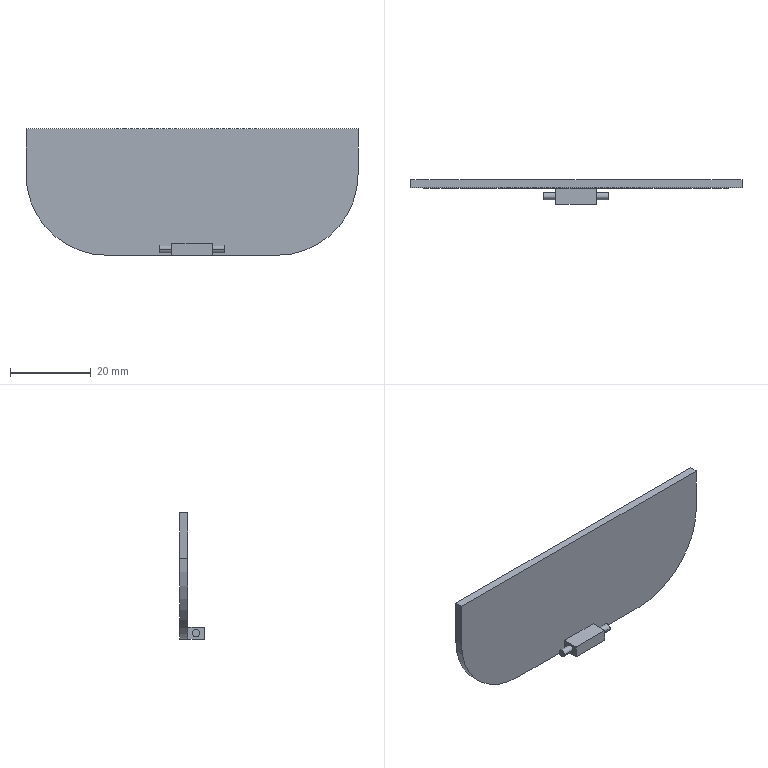Component | SolidWorks | WaterTankLid-2 | 1 solid | 18 faces | box 82.07 x 6 x 31.26 mm | volume 4923 mm3 | plane 12 | cylinder 6 | commonest cylinder face diameters 1.8 x4 40 x2
build123d program:
from build123d import *

# Parameters (mm, degrees)
BOSS_EXTRUDE1_DEPTH = 2
SKETCH6_W           = 10
SKETCH6_H           = 3
BOSS_EXTRUDE5_DEPTH = 4
SKETCH7_R           = 0.9
BOSS_EXTRUDE6_DEPTH = 3


with BuildPart() as part:
    # Sketch1 → Boss-Extrude1 (new body)
    with BuildSketch(Plane.XY):
        with BuildLine():
            ThreePointArc((-21.035, 58.449), (-35.177, 52.591), (-41.035, 38.449))
            Line((-41.035, 38.449), (-41.035, 27.187))
            Line((-41.035, 27.187), (41.035, 27.187))
            Line((41.035, 27.187), (41.035, 38.449))
            ThreePointArc((41.035, 38.449), (35.177, 52.591), (21.035, 58.449))
            Line((21.035, 58.449), (-21.035, 58.449))
        make_face()
    extrude(amount=BOSS_EXTRUDE1_DEPTH)

    # Sketch6 → Boss-Extrude5 (add)
    with BuildSketch(Plane.XY.offset(2)):
        with Locations((-0.0183, 56.949)):
            Rectangle(SKETCH6_W, SKETCH6_H)
    extrude(amount=BOSS_EXTRUDE5_DEPTH)

    # Sketch7 → Boss-Extrude6 (add)
    with BuildSketch(Plane.ZY.offset(5.018)):
        with Locations(Location((4, 56.949, 0), (0, 0, 180))):
            Circle(SKETCH7_R)
    boss_extrude6 = extrude(amount=BOSS_EXTRUDE6_DEPTH)

    # Mirror2: Boss-Extrude6 across plane
    add(boss_extrude6.mirror(Plane.ZY.offset(0.0183)))


solid = part.part

# Placed as in the assembly
solid = solid.moved(Location((-76.707, 22.584, 216.702), (90, 0, -180)))
STEP:
#1=COLOUR_RGB('',0.7922,0.8196,0.9333);
#2=FILL_AREA_STYLE_COLOUR('',#1);
#3=FILL_AREA_STYLE('',(#2));
#4=SURFACE_STYLE_FILL_AREA(#3);
#5=SURFACE_SIDE_STYLE('',(#4));
#6=SURFACE_STYLE_USAGE(.BOTH.,#5);
#7=PRESENTATION_STYLE_ASSIGNMENT((#6));
#8=CARTESIAN_POINT('',(-3.334,0.6962,6.289));
#9=VERTEX_POINT('',#8);
#10=CARTESIAN_POINT('',(-3.334,0.7671,6.289));
#11=VERTEX_POINT('',#10);
#12=CARTESIAN_POINT('',(-3.334,0.7317,6.289));
#13=DIRECTION('',(1.,0.,0.));
#14=DIRECTION('',(0.,-1.,0.));
#15=AXIS2_PLACEMENT_3D('',#12,#13,#14);
#16=CIRCLE('',#15,0.03543);
#17=EDGE_CURVE('',#9,#11,#16,.T.);
#18=ORIENTED_EDGE('',*,*,#17,.T.);
#19=CARTESIAN_POINT('',(-3.216,0.7671,6.289));
#20=VERTEX_POINT('',#19);
#21=CARTESIAN_POINT('',(-3.334,0.7671,6.289));
#22=DIRECTION('',(1.,0.,0.));
#23=VECTOR('',#22,39.37);
#24=LINE('',#21,#23);
#25=EDGE_CURVE('',#11,#20,#24,.T.);
#26=ORIENTED_EDGE('',*,*,#25,.T.);
#27=CARTESIAN_POINT('',(-3.216,0.6962,6.289));
#28=VERTEX_POINT('',#27);
#29=CARTESIAN_POINT('',(-3.216,0.7317,6.289));
#30=DIRECTION('',(1.,0.,0.));
#31=DIRECTION('',(0.,-1.,0.));
#32=AXIS2_PLACEMENT_3D('',#29,#30,#31);
#33=CIRCLE('',#32,0.03543);
#34=EDGE_CURVE('',#28,#20,#33,.T.);
#35=ORIENTED_EDGE('',*,*,#34,.F.);
#36=CARTESIAN_POINT('',(-3.334,0.6962,6.289));
#37=DIRECTION('',(1.,0.,0.));
#38=VECTOR('',#37,39.37);
#39=LINE('',#36,#38);
#40=EDGE_CURVE('',#9,#28,#39,.T.);
#41=ORIENTED_EDGE('',*,*,#40,.F.);
#42=EDGE_LOOP('',(#18,#26,#35,#41));
#43=FACE_OUTER_BOUND('',#42,.T.);
#44=CARTESIAN_POINT('',(-3.334,0.7317,6.289));
#45=DIRECTION('',(1.,0.,0.));
#46=DIRECTION('',(0.,-1.,0.));
#47=AXIS2_PLACEMENT_3D('',#44,#45,#46);
#48=CYLINDRICAL_SURFACE('',#47,0.03543);
#49=ADVANCED_FACE('',(#43),#48,.T.);
#50=CARTESIAN_POINT('',(-2.704,0.6962,6.289));
#51=VERTEX_POINT('',#50);
#52=CARTESIAN_POINT('',(-2.704,0.7671,6.289));
#53=VERTEX_POINT('',#52);
#54=CARTESIAN_POINT('',(-2.704,0.7317,6.289));
#55=DIRECTION('',(1.,0.,0.));
#56=DIRECTION('',(0.,-1.,0.));
#57=AXIS2_PLACEMENT_3D('',#54,#55,#56);
#58=CIRCLE('',#57,0.03543);
#59=EDGE_CURVE('',#51,#53,#58,.T.);
#60=ORIENTED_EDGE('',*,*,#59,.F.);
#61=CARTESIAN_POINT('',(-2.822,0.6962,6.289));
#62=VERTEX_POINT('',#61);
#63=CARTESIAN_POINT('',(-2.704,0.6962,6.289));
#64=DIRECTION('',(-1.,-0.,-0.));
#65=VECTOR('',#64,39.37);
#66=LINE('',#63,#65);
#67=EDGE_CURVE('',#51,#62,#66,.T.);
#68=ORIENTED_EDGE('',*,*,#67,.T.);
#69=CARTESIAN_POINT('',(-2.822,0.7671,6.289));
#70=VERTEX_POINT('',#69);
#71=CARTESIAN_POINT('',(-2.822,0.7317,6.289));
#72=DIRECTION('',(1.,0.,0.));
#73=DIRECTION('',(0.,1.,0.));
#74=AXIS2_PLACEMENT_3D('',#71,#72,#73);
#75=CIRCLE('',#74,0.03543);
#76=EDGE_CURVE('',#62,#70,#75,.T.);
#77=ORIENTED_EDGE('',*,*,#76,.T.);
#78=CARTESIAN_POINT('',(-2.704,0.7671,6.289));
#79=DIRECTION('',(-1.,-0.,-0.));
#80=VECTOR('',#79,39.37);
#81=LINE('',#78,#80);
#82=EDGE_CURVE('',#53,#70,#81,.T.);
#83=ORIENTED_EDGE('',*,*,#82,.F.);
#84=EDGE_LOOP('',(#60,#68,#77,#83));
#85=FACE_OUTER_BOUND('',#84,.T.);
#86=CARTESIAN_POINT('',(-2.704,0.7317,6.289));
#87=DIRECTION('',(-1.,-0.,-0.));
#88=DIRECTION('',(0.,1.,0.));
#89=AXIS2_PLACEMENT_3D('',#86,#87,#88);
#90=CYLINDRICAL_SURFACE('',#89,0.03543);
#91=ADVANCED_FACE('',(#85),#90,.T.);
#92=CARTESIAN_POINT('',(-4.636,0.8891,7.461));
#93=VERTEX_POINT('',#92);
#94=CARTESIAN_POINT('',(-4.636,0.8891,7.018));
#95=VERTEX_POINT('',#94);
#96=CARTESIAN_POINT('',(-4.636,0.8891,8.532));
#97=DIRECTION('',(0.,0.,-1.));
#98=VECTOR('',#97,39.37);
#99=LINE('',#96,#98);
#100=EDGE_CURVE('',#93,#95,#99,.T.);
#101=ORIENTED_EDGE('',*,*,#100,.T.);
#102=CARTESIAN_POINT('',(-4.636,0.8104,7.018));
#103=VERTEX_POINT('',#102);
#104=CARTESIAN_POINT('',(-4.636,0.8104,7.018));
#105=DIRECTION('',(-0.,1.,0.));
#106=VECTOR('',#105,39.37);
#107=LINE('',#104,#106);
#108=EDGE_CURVE('',#103,#95,#107,.T.);
#109=ORIENTED_EDGE('',*,*,#108,.F.);
#110=CARTESIAN_POINT('',(-4.636,0.8104,7.461));
#111=VERTEX_POINT('',#110);
#112=CARTESIAN_POINT('',(-4.636,0.8104,8.532));
#113=DIRECTION('',(0.,0.,-1.));
#114=VECTOR('',#113,39.37);
#115=LINE('',#112,#114);
#116=EDGE_CURVE('',#111,#103,#115,.T.);
#117=ORIENTED_EDGE('',*,*,#116,.F.);
#118=CARTESIAN_POINT('',(-4.636,0.8104,7.461));
#119=DIRECTION('',(-0.,1.,0.));
#120=VECTOR('',#119,39.37);
#121=LINE('',#118,#120);
#122=EDGE_CURVE('',#111,#93,#121,.T.);
#123=ORIENTED_EDGE('',*,*,#122,.T.);
#124=EDGE_LOOP('',(#101,#109,#117,#123));
#125=FACE_OUTER_BOUND('',#124,.T.);
#126=CARTESIAN_POINT('',(-4.636,0.8104,8.532));
#127=DIRECTION('',(1.,0.,0.));
#128=DIRECTION('',(0.,-1.,0.));
#129=AXIS2_PLACEMENT_3D('',#126,#127,#128);
#130=PLANE('',#129);
#131=ADVANCED_FACE('',(#125),#130,.F.);
#132=CARTESIAN_POINT('',(-3.848,0.8891,6.23));
#133=VERTEX_POINT('',#132);
#134=CARTESIAN_POINT('',(-3.848,0.8891,7.018));
#135=DIRECTION('',(0.,-1.,0.));
#136=DIRECTION('',(-1.,0.,0.));
#137=AXIS2_PLACEMENT_3D('',#134,#135,#136);
#138=CIRCLE('',#137,0.7874);
#139=EDGE_CURVE('',#95,#133,#138,.T.);
#140=ORIENTED_EDGE('',*,*,#139,.T.);
#141=CARTESIAN_POINT('',(-3.848,0.8104,6.23));
#142=VERTEX_POINT('',#141);
#143=CARTESIAN_POINT('',(-3.848,0.8104,6.23));
#144=DIRECTION('',(-0.,1.,0.));
#145=VECTOR('',#144,39.37);
#146=LINE('',#143,#145);
#147=EDGE_CURVE('',#142,#133,#146,.T.);
#148=ORIENTED_EDGE('',*,*,#147,.F.);
#149=CARTESIAN_POINT('',(-3.848,0.8104,7.018));
#150=DIRECTION('',(0.,-1.,0.));
#151=DIRECTION('',(-1.,0.,0.));
#152=AXIS2_PLACEMENT_3D('',#149,#150,#151);
#153=CIRCLE('',#152,0.7874);
#154=EDGE_CURVE('',#103,#142,#153,.T.);
#155=ORIENTED_EDGE('',*,*,#154,.F.);
#156=ORIENTED_EDGE('',*,*,#108,.T.);
#157=EDGE_LOOP('',(#140,#148,#155,#156));
#158=FACE_OUTER_BOUND('',#157,.T.);
#159=CARTESIAN_POINT('',(-3.848,0.8104,7.018));
#160=DIRECTION('',(-0.,1.,0.));
#161=DIRECTION('',(1.,0.,0.));
#162=AXIS2_PLACEMENT_3D('',#159,#160,#161);
#163=CYLINDRICAL_SURFACE('',#162,0.7874);
#164=ADVANCED_FACE('',(#158),#163,.T.);
#165=CARTESIAN_POINT('',(-2.192,0.8891,6.23));
#166=VERTEX_POINT('',#165);
#167=CARTESIAN_POINT('',(-3.02,0.8891,6.23));
#168=DIRECTION('',(1.,0.,0.));
#169=VECTOR('',#168,39.37);
#170=LINE('',#167,#169);
#171=EDGE_CURVE('',#133,#166,#170,.T.);
#172=ORIENTED_EDGE('',*,*,#171,.T.);
#173=CARTESIAN_POINT('',(-2.192,0.8104,6.23));
#174=VERTEX_POINT('',#173);
#175=CARTESIAN_POINT('',(-2.192,0.8104,6.23));
#176=DIRECTION('',(-0.,1.,0.));
#177=VECTOR('',#176,39.37);
#178=LINE('',#175,#177);
#179=EDGE_CURVE('',#174,#166,#178,.T.);
#180=ORIENTED_EDGE('',*,*,#179,.F.);
#181=CARTESIAN_POINT('',(-2.822,0.8104,6.23));
#182=VERTEX_POINT('',#181);
#183=CARTESIAN_POINT('',(-3.02,0.8104,6.23));
#184=DIRECTION('',(1.,0.,0.));
#185=VECTOR('',#184,39.37);
#186=LINE('',#183,#185);
#187=EDGE_CURVE('',#182,#174,#186,.T.);
#188=ORIENTED_EDGE('',*,*,#187,.F.);
#189=CARTESIAN_POINT('',(-2.822,0.6529,6.23));
#190=VERTEX_POINT('',#189);
#191=CARTESIAN_POINT('',(-2.822,0.6529,6.23));
#192=DIRECTION('',(-0.,1.,0.));
#193=VECTOR('',#192,39.37);
#194=LINE('',#191,#193);
#195=EDGE_CURVE('',#190,#182,#194,.T.);
#196=ORIENTED_EDGE('',*,*,#195,.F.);
#197=CARTESIAN_POINT('',(-3.216,0.6529,6.23));
#198=VERTEX_POINT('',#197);
#199=CARTESIAN_POINT('',(-2.822,0.6529,6.23));
#200=DIRECTION('',(1.,0.,-0.));
#201=VECTOR('',#200,39.37);
#202=LINE('',#199,#201);
#203=EDGE_CURVE('',#198,#190,#202,.T.);
#204=ORIENTED_EDGE('',*,*,#203,.F.);
#205=CARTESIAN_POINT('',(-3.216,0.8104,6.23));
#206=VERTEX_POINT('',#205);
#207=CARTESIAN_POINT('',(-3.216,0.6529,6.23));
#208=DIRECTION('',(-0.,1.,0.));
#209=VECTOR('',#208,39.37);
#210=LINE('',#207,#209);
#211=EDGE_CURVE('',#198,#206,#210,.T.);
#212=ORIENTED_EDGE('',*,*,#211,.T.);
#213=CARTESIAN_POINT('',(-3.02,0.8104,6.23));
#214=DIRECTION('',(1.,0.,0.));
#215=VECTOR('',#214,39.37);
#216=LINE('',#213,#215);
#217=EDGE_CURVE('',#142,#206,#216,.T.);
#218=ORIENTED_EDGE('',*,*,#217,.F.);
#219=ORIENTED_EDGE('',*,*,#147,.T.);
#220=EDGE_LOOP('',(#172,#180,#188,#196,#204,#212,#218,#219));
#221=FACE_OUTER_BOUND('',#220,.T.);
#222=CARTESIAN_POINT('',(-3.02,0.8104,6.23));
#223=DIRECTION('',(-0.,-0.,1.));
#224=DIRECTION('',(-0.,1.,0.));
#225=AXIS2_PLACEMENT_3D('',#222,#223,#224);
#226=PLANE('',#225);
#227=ADVANCED_FACE('',(#221),#226,.F.);
#228=CARTESIAN_POINT('',(-1.404,0.8891,7.018));
#229=VERTEX_POINT('',#228);
#230=CARTESIAN_POINT('',(-2.192,0.8891,7.018));
#231=DIRECTION('',(0.,-1.,0.));
#232=DIRECTION('',(-1.,0.,0.));
#233=AXIS2_PLACEMENT_3D('',#230,#231,#232);
#234=CIRCLE('',#233,0.7874);
#235=EDGE_CURVE('',#166,#229,#234,.T.);
#236=ORIENTED_EDGE('',*,*,#235,.T.);
#237=CARTESIAN_POINT('',(-1.404,0.8104,7.018));
#238=VERTEX_POINT('',#237);
#239=CARTESIAN_POINT('',(-1.404,0.8104,7.018));
#240=DIRECTION('',(-0.,1.,0.));
#241=VECTOR('',#240,39.37);
#242=LINE('',#239,#241);
#243=EDGE_CURVE('',#238,#229,#242,.T.);
#244=ORIENTED_EDGE('',*,*,#243,.F.);
#245=CARTESIAN_POINT('',(-2.192,0.8104,7.018));
#246=DIRECTION('',(0.,-1.,0.));
#247=DIRECTION('',(-1.,0.,0.));
#248=AXIS2_PLACEMENT_3D('',#245,#246,#247);
#249=CIRCLE('',#248,0.7874);
#250=EDGE_CURVE('',#174,#238,#249,.T.);
#251=ORIENTED_EDGE('',*,*,#250,.F.);
#252=ORIENTED_EDGE('',*,*,#179,.T.);
#253=EDGE_LOOP('',(#236,#244,#251,#252));
#254=FACE_OUTER_BOUND('',#253,.T.);
#255=CARTESIAN_POINT('',(-2.192,0.8104,7.018));
#256=DIRECTION('',(-0.,1.,0.));
#257=DIRECTION('',(1.,0.,0.));
#258=AXIS2_PLACEMENT_3D('',#255,#256,#257);
#259=CYLINDRICAL_SURFACE('',#258,0.7874);
#260=ADVANCED_FACE('',(#254),#259,.T.);
#261=CARTESIAN_POINT('',(-1.404,0.8891,7.461));
#262=VERTEX_POINT('',#261);
#263=CARTESIAN_POINT('',(-1.404,0.8891,8.532));
#264=DIRECTION('',(-0.,0.,1.));
#265=VECTOR('',#264,39.37);
#266=LINE('',#263,#265);
#267=EDGE_CURVE('',#229,#262,#266,.T.);
#268=ORIENTED_EDGE('',*,*,#267,.T.);
#269=CARTESIAN_POINT('',(-1.404,0.8104,7.461));
#270=VERTEX_POINT('',#269);
#271=CARTESIAN_POINT('',(-1.404,0.8104,7.461));
#272=DIRECTION('',(-0.,1.,0.));
#273=VECTOR('',#272,39.37);
#274=LINE('',#271,#273);
#275=EDGE_CURVE('',#270,#262,#274,.T.);
#276=ORIENTED_EDGE('',*,*,#275,.F.);
#277=CARTESIAN_POINT('',(-1.404,0.8104,8.532));
#278=DIRECTION('',(-0.,0.,1.));
#279=VECTOR('',#278,39.37);
#280=LINE('',#277,#279);
#281=EDGE_CURVE('',#238,#270,#280,.T.);
#282=ORIENTED_EDGE('',*,*,#281,.F.);
#283=ORIENTED_EDGE('',*,*,#243,.T.);
#284=EDGE_LOOP('',(#268,#276,#282,#283));
#285=FACE_OUTER_BOUND('',#284,.T.);
#286=CARTESIAN_POINT('',(-1.404,0.8104,8.532));
#287=DIRECTION('',(-1.,-0.,-0.));
#288=DIRECTION('',(-0.,1.,0.));
#289=AXIS2_PLACEMENT_3D('',#286,#287,#288);
#290=PLANE('',#289);
#291=ADVANCED_FACE('',(#285),#290,.F.);
#292=CARTESIAN_POINT('',(-3.02,0.8891,7.461));
#293=DIRECTION('',(-1.,-0.,-0.));
#294=VECTOR('',#293,39.37);
#295=LINE('',#292,#294);
#296=EDGE_CURVE('',#262,#93,#295,.T.);
#297=ORIENTED_EDGE('',*,*,#296,.T.);
#298=ORIENTED_EDGE('',*,*,#122,.F.);
#299=CARTESIAN_POINT('',(-3.02,0.8104,7.461));
#300=DIRECTION('',(-1.,-0.,-0.));
#301=VECTOR('',#300,39.37);
#302=LINE('',#299,#301);
#303=EDGE_CURVE('',#270,#111,#302,.T.);
#304=ORIENTED_EDGE('',*,*,#303,.F.);
#305=ORIENTED_EDGE('',*,*,#275,.T.);
#306=EDGE_LOOP('',(#297,#298,#304,#305));
#307=FACE_OUTER_BOUND('',#306,.T.);
#308=CARTESIAN_POINT('',(-3.02,0.8104,7.461));
#309=DIRECTION('',(0.,-0.,-1.));
#310=DIRECTION('',(1.,0.,0.));
#311=AXIS2_PLACEMENT_3D('',#308,#309,#310);
#312=PLANE('',#311);
#313=ADVANCED_FACE('',(#307),#312,.F.);
#314=CARTESIAN_POINT('',(-2.822,0.8104,6.349));
#315=VERTEX_POINT('',#314);
#316=CARTESIAN_POINT('',(-2.822,0.8104,6.23));
#317=DIRECTION('',(-0.,0.,1.));
#318=VECTOR('',#317,39.37);
#319=LINE('',#316,#318);
#320=EDGE_CURVE('',#182,#315,#319,.T.);
#321=ORIENTED_EDGE('',*,*,#320,.F.);
#322=ORIENTED_EDGE('',*,*,#187,.T.);
#323=ORIENTED_EDGE('',*,*,#250,.T.);
#324=ORIENTED_EDGE('',*,*,#281,.T.);
#325=ORIENTED_EDGE('',*,*,#303,.T.);
#326=ORIENTED_EDGE('',*,*,#116,.T.);
#327=ORIENTED_EDGE('',*,*,#154,.T.);
#328=ORIENTED_EDGE('',*,*,#217,.T.);
#329=CARTESIAN_POINT('',(-3.216,0.8104,6.349));
#330=VERTEX_POINT('',#329);
#331=CARTESIAN_POINT('',(-3.216,0.8104,6.23));
#332=DIRECTION('',(0.,0.,-1.));
#333=VECTOR('',#332,39.37);
#334=LINE('',#331,#333);
#335=EDGE_CURVE('',#330,#206,#334,.T.);
#336=ORIENTED_EDGE('',*,*,#335,.F.);
#337=CARTESIAN_POINT('',(-2.822,0.8104,6.349));
#338=DIRECTION('',(-1.,-0.,-0.));
#339=VECTOR('',#338,39.37);
#340=LINE('',#337,#339);
#341=EDGE_CURVE('',#315,#330,#340,.T.);
#342=ORIENTED_EDGE('',*,*,#341,.F.);
#343=EDGE_LOOP('',(#321,#322,#323,#324,#325,#326,#327,#328,#336,#342));
#344=FACE_OUTER_BOUND('',#343,.T.);
#345=CARTESIAN_POINT('',(-3.02,0.8104,8.532));
#346=DIRECTION('',(0.,-1.,-0.));
#347=DIRECTION('',(-1.,-0.,-0.));
#348=AXIS2_PLACEMENT_3D('',#345,#346,#347);
#349=PLANE('',#348);
#350=ADVANCED_FACE('',(#344),#349,.T.);
#351=ORIENTED_EDGE('',*,*,#100,.F.);
#352=ORIENTED_EDGE('',*,*,#296,.F.);
#353=ORIENTED_EDGE('',*,*,#267,.F.);
#354=ORIENTED_EDGE('',*,*,#235,.F.);
#355=ORIENTED_EDGE('',*,*,#171,.F.);
#356=ORIENTED_EDGE('',*,*,#139,.F.);
#357=EDGE_LOOP('',(#351,#352,#353,#354,#355,#356));
#358=FACE_OUTER_BOUND('',#357,.T.);
#359=CARTESIAN_POINT('',(-3.02,0.8891,8.532));
#360=DIRECTION('',(0.,-1.,-0.));
#361=DIRECTION('',(-1.,-0.,-0.));
#362=AXIS2_PLACEMENT_3D('',#359,#360,#361);
#363=PLANE('',#362);
#364=ADVANCED_FACE('',(#358),#363,.F.);
#365=CARTESIAN_POINT('',(-2.822,0.7317,6.289));
#366=DIRECTION('',(1.,0.,0.));
#367=DIRECTION('',(0.,1.,0.));
#368=AXIS2_PLACEMENT_3D('',#365,#366,#367);
#369=CIRCLE('',#368,0.03543);
#370=EDGE_CURVE('',#70,#62,#369,.T.);
#371=ORIENTED_EDGE('',*,*,#370,.F.);
#372=ORIENTED_EDGE('',*,*,#76,.F.);
#373=EDGE_LOOP('',(#371,#372));
#374=FACE_BOUND('',#373,.T.);
#375=ORIENTED_EDGE('',*,*,#320,.T.);
#376=CARTESIAN_POINT('',(-2.822,0.6529,6.349));
#377=VERTEX_POINT('',#376);
#378=CARTESIAN_POINT('',(-2.822,0.6529,6.349));
#379=DIRECTION('',(-0.,1.,0.));
#380=VECTOR('',#379,39.37);
#381=LINE('',#378,#380);
#382=EDGE_CURVE('',#377,#315,#381,.T.);
#383=ORIENTED_EDGE('',*,*,#382,.F.);
#384=CARTESIAN_POINT('',(-2.822,0.6529,6.23));
#385=DIRECTION('',(-0.,0.,1.));
#386=VECTOR('',#385,39.37);
#387=LINE('',#384,#386);
#388=EDGE_CURVE('',#190,#377,#387,.T.);
#389=ORIENTED_EDGE('',*,*,#388,.F.);
#390=ORIENTED_EDGE('',*,*,#195,.T.);
#391=EDGE_LOOP('',(#375,#383,#389,#390));
#392=FACE_OUTER_BOUND('',#391,.T.);
#393=CARTESIAN_POINT('',(-2.822,0.6529,6.23));
#394=DIRECTION('',(-1.,-0.,-0.));
#395=DIRECTION('',(-0.,1.,0.));
#396=AXIS2_PLACEMENT_3D('',#393,#394,#395);
#397=PLANE('',#396);
#398=ADVANCED_FACE('',(#374,#392),#397,.F.);
#399=ORIENTED_EDGE('',*,*,#341,.T.);
#400=CARTESIAN_POINT('',(-3.216,0.6529,6.349));
#401=VERTEX_POINT('',#400);
#402=CARTESIAN_POINT('',(-3.216,0.6529,6.349));
#403=DIRECTION('',(-0.,1.,0.));
#404=VECTOR('',#403,39.37);
#405=LINE('',#402,#404);
#406=EDGE_CURVE('',#401,#330,#405,.T.);
#407=ORIENTED_EDGE('',*,*,#406,.F.);
#408=CARTESIAN_POINT('',(-2.822,0.6529,6.349));
#409=DIRECTION('',(-1.,-0.,-0.));
#410=VECTOR('',#409,39.37);
#411=LINE('',#408,#410);
#412=EDGE_CURVE('',#377,#401,#411,.T.);
#413=ORIENTED_EDGE('',*,*,#412,.F.);
#414=ORIENTED_EDGE('',*,*,#382,.T.);
#415=EDGE_LOOP('',(#399,#407,#413,#414));
#416=FACE_OUTER_BOUND('',#415,.T.);
#417=CARTESIAN_POINT('',(-2.822,0.6529,6.349));
#418=DIRECTION('',(0.,0.,-1.));
#419=DIRECTION('',(0.,-1.,0.));
#420=AXIS2_PLACEMENT_3D('',#417,#418,#419);
#421=PLANE('',#420);
#422=ADVANCED_FACE('',(#416),#421,.F.);
#423=ORIENTED_EDGE('',*,*,#34,.T.);
#424=CARTESIAN_POINT('',(-3.216,0.7317,6.289));
#425=DIRECTION('',(1.,0.,0.));
#426=DIRECTION('',(0.,-1.,0.));
#427=AXIS2_PLACEMENT_3D('',#424,#425,#426);
#428=CIRCLE('',#427,0.03543);
#429=EDGE_CURVE('',#20,#28,#428,.T.);
#430=ORIENTED_EDGE('',*,*,#429,.T.);
#431=EDGE_LOOP('',(#423,#430));
#432=FACE_BOUND('',#431,.T.);
#433=ORIENTED_EDGE('',*,*,#335,.T.);
#434=ORIENTED_EDGE('',*,*,#211,.F.);
#435=CARTESIAN_POINT('',(-3.216,0.6529,6.23));
#436=DIRECTION('',(0.,0.,-1.));
#437=VECTOR('',#436,39.37);
#438=LINE('',#435,#437);
#439=EDGE_CURVE('',#401,#198,#438,.T.);
#440=ORIENTED_EDGE('',*,*,#439,.F.);
#441=ORIENTED_EDGE('',*,*,#406,.T.);
#442=EDGE_LOOP('',(#433,#434,#440,#441));
#443=FACE_OUTER_BOUND('',#442,.T.);
#444=CARTESIAN_POINT('',(-3.216,0.6529,6.23));
#445=DIRECTION('',(1.,0.,0.));
#446=DIRECTION('',(0.,-1.,0.));
#447=AXIS2_PLACEMENT_3D('',#444,#445,#446);
#448=PLANE('',#447);
#449=ADVANCED_FACE('',(#432,#443),#448,.F.);
#450=ORIENTED_EDGE('',*,*,#388,.T.);
#451=ORIENTED_EDGE('',*,*,#412,.T.);
#452=ORIENTED_EDGE('',*,*,#439,.T.);
#453=ORIENTED_EDGE('',*,*,#203,.T.);
#454=EDGE_LOOP('',(#450,#451,#452,#453));
#455=FACE_OUTER_BOUND('',#454,.T.);
#456=CARTESIAN_POINT('',(-3.02,0.6529,8.532));
#457=DIRECTION('',(0.,-1.,-0.));
#458=DIRECTION('',(-1.,-0.,-0.));
#459=AXIS2_PLACEMENT_3D('',#456,#457,#458);
#460=PLANE('',#459);
#461=ADVANCED_FACE('',(#455),#460,.T.);
#462=ORIENTED_EDGE('',*,*,#67,.F.);
#463=CARTESIAN_POINT('',(-2.704,0.7317,6.289));
#464=DIRECTION('',(1.,0.,0.));
#465=DIRECTION('',(0.,-1.,0.));
#466=AXIS2_PLACEMENT_3D('',#463,#464,#465);
#467=CIRCLE('',#466,0.03543);
#468=EDGE_CURVE('',#53,#51,#467,.T.);
#469=ORIENTED_EDGE('',*,*,#468,.F.);
#470=ORIENTED_EDGE('',*,*,#82,.T.);
#471=ORIENTED_EDGE('',*,*,#370,.T.);
#472=EDGE_LOOP('',(#462,#469,#470,#471));
#473=FACE_OUTER_BOUND('',#472,.T.);
#474=CARTESIAN_POINT('',(-2.704,0.7317,6.289));
#475=DIRECTION('',(-1.,-0.,-0.));
#476=DIRECTION('',(0.,1.,0.));
#477=AXIS2_PLACEMENT_3D('',#474,#475,#476);
#478=CYLINDRICAL_SURFACE('',#477,0.03543);
#479=ADVANCED_FACE('',(#473),#478,.T.);
#480=ORIENTED_EDGE('',*,*,#468,.T.);
#481=ORIENTED_EDGE('',*,*,#59,.T.);
#482=EDGE_LOOP('',(#480,#481));
#483=FACE_OUTER_BOUND('',#482,.T.);
#484=CARTESIAN_POINT('',(-2.704,0.7317,6.289));
#485=DIRECTION('',(1.,0.,0.));
#486=DIRECTION('',(0.,-1.,0.));
#487=AXIS2_PLACEMENT_3D('',#484,#485,#486);
#488=PLANE('',#487);
#489=ADVANCED_FACE('',(#483),#488,.T.);
#490=ORIENTED_EDGE('',*,*,#25,.F.);
#491=CARTESIAN_POINT('',(-3.334,0.7317,6.289));
#492=DIRECTION('',(1.,0.,0.));
#493=DIRECTION('',(0.,-1.,0.));
#494=AXIS2_PLACEMENT_3D('',#491,#492,#493);
#495=CIRCLE('',#494,0.03543);
#496=EDGE_CURVE('',#11,#9,#495,.T.);
#497=ORIENTED_EDGE('',*,*,#496,.T.);
#498=ORIENTED_EDGE('',*,*,#40,.T.);
#499=ORIENTED_EDGE('',*,*,#429,.F.);
#500=EDGE_LOOP('',(#490,#497,#498,#499));
#501=FACE_OUTER_BOUND('',#500,.T.);
#502=CARTESIAN_POINT('',(-3.334,0.7317,6.289));
#503=DIRECTION('',(1.,0.,0.));
#504=DIRECTION('',(0.,-1.,0.));
#505=AXIS2_PLACEMENT_3D('',#502,#503,#504);
#506=CYLINDRICAL_SURFACE('',#505,0.03543);
#507=ADVANCED_FACE('',(#501),#506,.T.);
#508=ORIENTED_EDGE('',*,*,#17,.F.);
#509=ORIENTED_EDGE('',*,*,#496,.F.);
#510=EDGE_LOOP('',(#508,#509));
#511=FACE_OUTER_BOUND('',#510,.T.);
#512=CARTESIAN_POINT('',(-3.334,0.7317,6.289));
#513=DIRECTION('',(-1.,-0.,-0.));
#514=DIRECTION('',(0.,-1.,0.));
#515=AXIS2_PLACEMENT_3D('',#512,#513,#514);
#516=PLANE('',#515);
#517=ADVANCED_FACE('',(#511),#516,.T.);
#518=CLOSED_SHELL('',(#49,#91,#131,#164,#227,#260,#291,#313,#350,#364,#398,#422,#449,#461,#479,#489,#507,#517));
#519=MANIFOLD_SOLID_BREP('',#518);
#520=STYLED_ITEM('',(#7),#519);
#521=PRESENTATION_LAYER_ASSIGNMENT('','',(#520));
#522=CARTESIAN_POINT('',(0.,0.,0.));
#523=DIRECTION('',(0.,0.,1.));
#524=DIRECTION('',(1.,0.,0.));
#525=AXIS2_PLACEMENT_3D('',#522,#523,#524);
#526=(LENGTH_UNIT()NAMED_UNIT(*)SI_UNIT($,.METRE.));
#527=LENGTH_MEASURE_WITH_UNIT(LENGTH_MEASURE(0.0254),#526);
#528=DIMENSIONAL_EXPONENTS(1.,0.,0.,0.,0.,0.,0.);
#529=(CONVERSION_BASED_UNIT('',#527)LENGTH_UNIT()NAMED_UNIT(#528));
#530=UNCERTAINTY_MEASURE_WITH_UNIT(LENGTH_MEASURE(0.00001),#529,'','');
#531=(NAMED_UNIT(*)PLANE_ANGLE_UNIT()SI_UNIT($,.RADIAN.));
#532=(NAMED_UNIT(*)SI_UNIT($,.STERADIAN.)SOLID_ANGLE_UNIT());
#533=(GEOMETRIC_REPRESENTATION_CONTEXT(3)GLOBAL_UNCERTAINTY_ASSIGNED_CONTEXT((#530))GLOBAL_UNIT_ASSIGNED_CONTEXT((#529,#531,#532))REPRESENTATION_CONTEXT('',''));
#534=ADVANCED_BREP_SHAPE_REPRESENTATION('',(#519,#525),#533);
#535=(LENGTH_UNIT()NAMED_UNIT(*)SI_UNIT($,.METRE.));
#536=LENGTH_MEASURE_WITH_UNIT(LENGTH_MEASURE(0.0254),#535);
#537=DIMENSIONAL_EXPONENTS(1.,0.,0.,0.,0.,0.,0.);
#538=(CONVERSION_BASED_UNIT('',#536)LENGTH_UNIT()NAMED_UNIT(#537));
#539=UNCERTAINTY_MEASURE_WITH_UNIT(LENGTH_MEASURE(0.00001),#538,'','');
#540=(NAMED_UNIT(*)PLANE_ANGLE_UNIT()SI_UNIT($,.RADIAN.));
#541=(NAMED_UNIT(*)SI_UNIT($,.STERADIAN.)SOLID_ANGLE_UNIT());
#542=(GEOMETRIC_REPRESENTATION_CONTEXT(3)GLOBAL_UNCERTAINTY_ASSIGNED_CONTEXT((#539))GLOBAL_UNIT_ASSIGNED_CONTEXT((#538,#540,#541))REPRESENTATION_CONTEXT('',''));
#543=MECHANICAL_DESIGN_GEOMETRIC_PRESENTATION_REPRESENTATION('',(#520),#542);